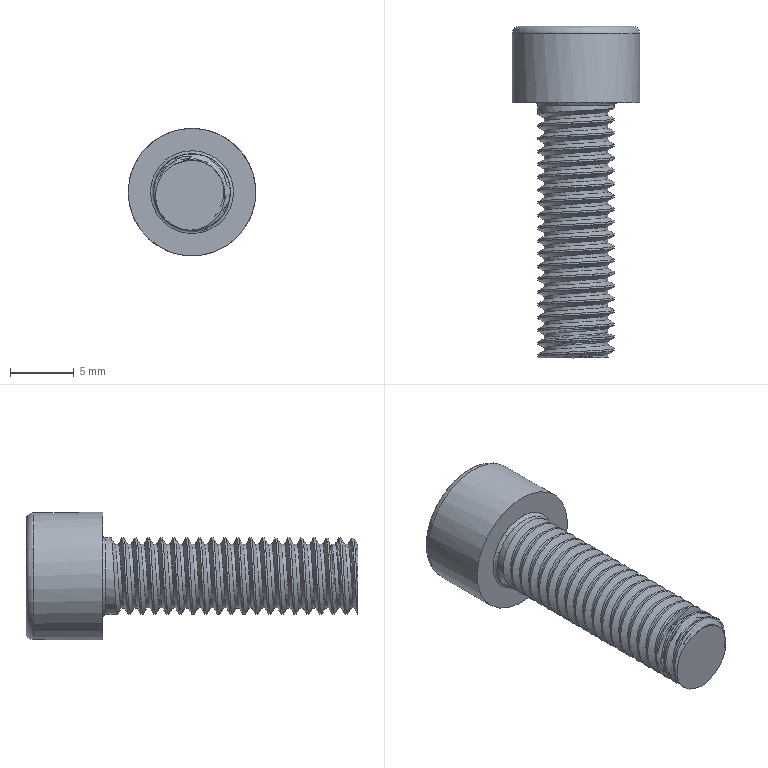Component | NX | M6X20_INT_3 | 1 solid | 30 faces | volume 868 mm3 | plane 16 | cone 7 | cylinder 3 | torus 2 | spline 2 | commonest cylinder face diameters 6 x1 10 x1 5 x1